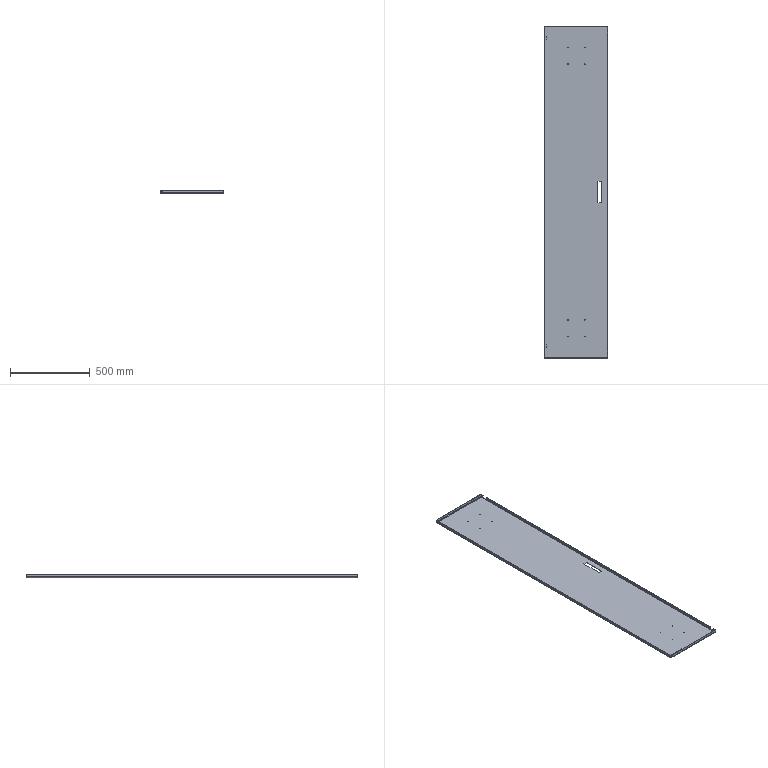Component | SolidWorks | RightRearDoor-1_RearDoor-1 | 1 solid | 86 faces | volume 1805995 mm3 | plane 42 | cylinder 36 | spline 8 | commonest cylinder face diameters 5 x20 3.2 x8 7 x4 11 x4 | material Malleable Cast Iron